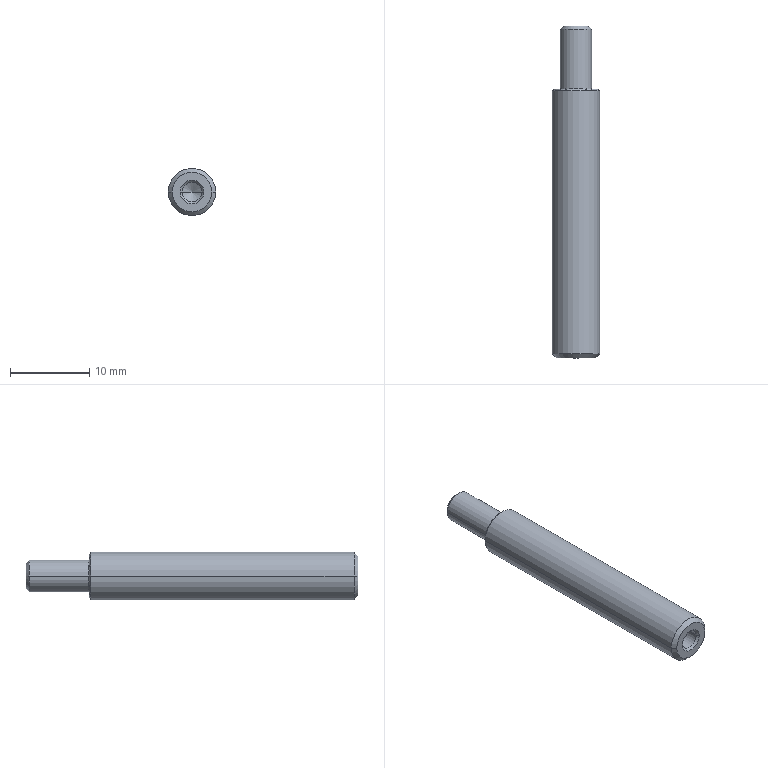Component | SolidWorks | SGE14-D6-L34-F8-B6-P4-N3-1 | 1 solid | 21 faces | box 6 x 42 x 6 mm | volume 1025 mm3 | cone 10 | cylinder 6 | plane 3 | torus 2 | commonest cylinder face diameters 2.459 x2 6 x2 4 x2
build123d program:
from build123d import *


with BuildPart() as part:
    # Sketch1 → Revolve1 (revolve)
    with BuildSketch(Plane(origin=(0, 0, 0), x_dir=(0, 0, -1), z_dir=(1, 0, 0)), mode=Mode.PRIVATE) as revolve1_sk:
        with BuildLine():
            Line((0, 0), (0, 2.5))
            Line((0, 2.5), (0.5, 3))
            Line((0.5, 3), (33.8, 3))
            Line((33.8, 3), (34, 2.8))
            Line((34, 2.8), (34, 2.1))
            ThreePointArc((34, 2.1), (34.029, 2.029), (34.1, 2))
            Line((34.1, 2), (41.571, 2))
            Line((41.571, 2), (42, 1.571))
            Line((42, 1.571), (42, 0))
            Line((42, 0), (0, 0))
        make_face()
    revolve(revolve1_sk.sketch.rotate(Axis((0, 0, -42), (0, 0, 1)), 270), axis=Axis((0, 0, -42), (0, 0, 1)))

    # Sketch2 → Cut-Revolve1 (revolve, cut)
    with BuildSketch(Plane(origin=(0, 0, 0), x_dir=(0, 0, -1), z_dir=(1, 0, 0)), mode=Mode.PRIVATE) as cut_revolve1_sk:
        Polygon((0, 0), (0, 1.5), (0.2705, 1.23), (6.656, 1.23), (7.366, 0), align=None)
    revolve(cut_revolve1_sk.sketch.rotate(Axis((0, 0, -7.366), (0, 0, 1)), 270), axis=Axis((0, 0, -7.366), (0, 0, 1)), mode=Mode.SUBTRACT)


solid = part.part

# Placed as in the assembly
solid = solid.moved(Location((-57.536, 39.25, 217.788), (90, 0, 0)))
STEP:
#1=COLOUR_RGB('',0.7922,0.8196,0.9333);
#2=FILL_AREA_STYLE_COLOUR('',#1);
#3=FILL_AREA_STYLE('',(#2));
#4=SURFACE_STYLE_FILL_AREA(#3);
#5=SURFACE_SIDE_STYLE('',(#4));
#6=SURFACE_STYLE_USAGE(.BOTH.,#5);
#7=PRESENTATION_STYLE_ASSIGNMENT((#6));
#8=CARTESIAN_POINT('',(-2.265,1.835,8.574));
#9=VERTEX_POINT('',#8);
#10=CARTESIAN_POINT('',(-2.217,1.807,8.574));
#11=VERTEX_POINT('',#10);
#12=CARTESIAN_POINT('',(-2.265,1.835,8.574));
#13=DIRECTION('',(0.866,-0.5,-0.));
#14=VECTOR('',#13,39.37);
#15=LINE('',#12,#14);
#16=EDGE_CURVE('',#9,#11,#15,.T.);
#17=ORIENTED_EDGE('',*,*,#16,.F.);
#18=CARTESIAN_POINT('',(-2.314,1.807,8.574));
#19=VERTEX_POINT('',#18);
#20=CARTESIAN_POINT('',(-2.265,1.835,8.574));
#21=DIRECTION('',(-0.866,-0.5,0.));
#22=VECTOR('',#21,39.37);
#23=LINE('',#20,#22);
#24=EDGE_CURVE('',#9,#19,#23,.T.);
#25=ORIENTED_EDGE('',*,*,#24,.T.);
#26=CARTESIAN_POINT('',(-2.265,1.807,8.574));
#27=DIRECTION('',(0.,-1.,-0.));
#28=DIRECTION('',(1.,0.,0.));
#29=AXIS2_PLACEMENT_3D('',#26,#27,#28);
#30=CIRCLE('',#29,0.04841);
#31=EDGE_CURVE('',#19,#11,#30,.T.);
#32=ORIENTED_EDGE('',*,*,#31,.T.);
#33=EDGE_LOOP('',(#17,#25,#32));
#34=FACE_OUTER_BOUND('',#33,.T.);
#35=CARTESIAN_POINT('',(-2.265,-37.535,8.574));
#36=DIRECTION('',(0.,-1.,-0.));
#37=DIRECTION('',(1.,0.,-0.));
#38=AXIS2_PLACEMENT_3D('',#35,#36,#37);
#39=CONICAL_SURFACE('',#38,68.191,1.047);
#40=ADVANCED_FACE('',(#34),#39,.F.);
#41=ORIENTED_EDGE('',*,*,#31,.F.);
#42=CARTESIAN_POINT('',(-2.314,1.556,8.574));
#43=VERTEX_POINT('',#42);
#44=CARTESIAN_POINT('',(-2.314,1.835,8.574));
#45=DIRECTION('',(0.,-1.,-0.));
#46=VECTOR('',#45,39.37);
#47=LINE('',#44,#46);
#48=EDGE_CURVE('',#19,#43,#47,.T.);
#49=ORIENTED_EDGE('',*,*,#48,.T.);
#50=CARTESIAN_POINT('',(-2.217,1.556,8.574));
#51=VERTEX_POINT('',#50);
#52=CARTESIAN_POINT('',(-2.265,1.556,8.574));
#53=DIRECTION('',(0.,-1.,-0.));
#54=DIRECTION('',(1.,0.,0.));
#55=AXIS2_PLACEMENT_3D('',#52,#53,#54);
#56=CIRCLE('',#55,0.04841);
#57=EDGE_CURVE('',#43,#51,#56,.T.);
#58=ORIENTED_EDGE('',*,*,#57,.T.);
#59=CARTESIAN_POINT('',(-2.217,1.835,8.574));
#60=DIRECTION('',(0.,-1.,-0.));
#61=VECTOR('',#60,39.37);
#62=LINE('',#59,#61);
#63=EDGE_CURVE('',#11,#51,#62,.T.);
#64=ORIENTED_EDGE('',*,*,#63,.F.);
#65=EDGE_LOOP('',(#41,#49,#58,#64));
#66=FACE_OUTER_BOUND('',#65,.T.);
#67=CARTESIAN_POINT('',(-2.265,1.835,8.574));
#68=DIRECTION('',(0.,-1.,-0.));
#69=DIRECTION('',(1.,0.,0.));
#70=AXIS2_PLACEMENT_3D('',#67,#68,#69);
#71=CYLINDRICAL_SURFACE('',#70,0.04841);
#72=ADVANCED_FACE('',(#66),#71,.F.);
#73=ORIENTED_EDGE('',*,*,#57,.F.);
#74=CARTESIAN_POINT('',(-2.324,1.545,8.574));
#75=VERTEX_POINT('',#74);
#76=CARTESIAN_POINT('',(-2.314,1.556,8.574));
#77=DIRECTION('',(-0.7071,-0.7071,0.));
#78=VECTOR('',#77,39.37);
#79=LINE('',#76,#78);
#80=EDGE_CURVE('',#43,#75,#79,.T.);
#81=ORIENTED_EDGE('',*,*,#80,.T.);
#82=CARTESIAN_POINT('',(-2.206,1.545,8.574));
#83=VERTEX_POINT('',#82);
#84=CARTESIAN_POINT('',(-2.265,1.545,8.574));
#85=DIRECTION('',(0.,-1.,-0.));
#86=DIRECTION('',(1.,0.,0.));
#87=AXIS2_PLACEMENT_3D('',#84,#85,#86);
#88=CIRCLE('',#87,0.05906);
#89=EDGE_CURVE('',#75,#83,#88,.T.);
#90=ORIENTED_EDGE('',*,*,#89,.T.);
#91=CARTESIAN_POINT('',(-2.217,1.556,8.574));
#92=DIRECTION('',(0.7071,-0.7071,-0.));
#93=VECTOR('',#92,39.37);
#94=LINE('',#91,#93);
#95=EDGE_CURVE('',#51,#83,#94,.T.);
#96=ORIENTED_EDGE('',*,*,#95,.F.);
#97=EDGE_LOOP('',(#73,#81,#90,#96));
#98=FACE_OUTER_BOUND('',#97,.T.);
#99=CARTESIAN_POINT('',(-2.265,1.556,8.574));
#100=DIRECTION('',(0.,-1.,-0.));
#101=DIRECTION('',(1.,0.,0.));
#102=AXIS2_PLACEMENT_3D('',#99,#100,#101);
#103=CONICAL_SURFACE('',#102,0.04841,0.7854);
#104=ADVANCED_FACE('',(#98),#103,.F.);
#105=CARTESIAN_POINT('',(-2.167,1.545,8.574));
#106=VERTEX_POINT('',#105);
#107=CARTESIAN_POINT('',(-2.364,1.545,8.574));
#108=VERTEX_POINT('',#107);
#109=CARTESIAN_POINT('',(-2.265,1.545,8.574));
#110=DIRECTION('',(0.,-1.,-0.));
#111=DIRECTION('',(1.,0.,0.));
#112=AXIS2_PLACEMENT_3D('',#109,#110,#111);
#113=CIRCLE('',#112,0.09843);
#114=EDGE_CURVE('',#106,#108,#113,.T.);
#115=ORIENTED_EDGE('',*,*,#114,.F.);
#116=CARTESIAN_POINT('',(-2.147,1.565,8.574));
#117=VERTEX_POINT('',#116);
#118=CARTESIAN_POINT('',(-2.147,1.565,8.574));
#119=DIRECTION('',(0.7071,0.7071,0.));
#120=VECTOR('',#119,39.37);
#121=LINE('',#118,#120);
#122=EDGE_CURVE('',#106,#117,#121,.T.);
#123=ORIENTED_EDGE('',*,*,#122,.T.);
#124=CARTESIAN_POINT('',(-2.383,1.565,8.574));
#125=VERTEX_POINT('',#124);
#126=CARTESIAN_POINT('',(-2.265,1.565,8.574));
#127=DIRECTION('',(0.,-1.,-0.));
#128=DIRECTION('',(1.,0.,0.));
#129=AXIS2_PLACEMENT_3D('',#126,#127,#128);
#130=CIRCLE('',#129,0.1181);
#131=EDGE_CURVE('',#117,#125,#130,.T.);
#132=ORIENTED_EDGE('',*,*,#131,.T.);
#133=CARTESIAN_POINT('',(-2.383,1.565,8.574));
#134=DIRECTION('',(-0.7071,0.7071,0.));
#135=VECTOR('',#134,39.37);
#136=LINE('',#133,#135);
#137=EDGE_CURVE('',#108,#125,#136,.T.);
#138=ORIENTED_EDGE('',*,*,#137,.F.);
#139=EDGE_LOOP('',(#115,#123,#132,#138));
#140=FACE_OUTER_BOUND('',#139,.T.);
#141=CARTESIAN_POINT('',(-2.265,1.565,8.574));
#142=DIRECTION('',(-0.,1.,0.));
#143=DIRECTION('',(-1.,0.,0.));
#144=AXIS2_PLACEMENT_3D('',#141,#142,#143);
#145=CONICAL_SURFACE('',#144,0.1181,0.7854);
#146=ADVANCED_FACE('',(#140),#145,.T.);
#147=CARTESIAN_POINT('',(-2.147,2.876,8.574));
#148=VERTEX_POINT('',#147);
#149=CARTESIAN_POINT('',(-2.383,2.876,8.574));
#150=VERTEX_POINT('',#149);
#151=CARTESIAN_POINT('',(-2.265,2.876,8.574));
#152=DIRECTION('',(0.,-1.,-0.));
#153=DIRECTION('',(1.,0.,0.));
#154=AXIS2_PLACEMENT_3D('',#151,#152,#153);
#155=CIRCLE('',#154,0.1181);
#156=EDGE_CURVE('',#148,#150,#155,.T.);
#157=ORIENTED_EDGE('',*,*,#156,.T.);
#158=CARTESIAN_POINT('',(-2.383,3.199,8.574));
#159=DIRECTION('',(0.,-1.,-0.));
#160=VECTOR('',#159,39.37);
#161=LINE('',#158,#160);
#162=EDGE_CURVE('',#150,#125,#161,.T.);
#163=ORIENTED_EDGE('',*,*,#162,.T.);
#164=ORIENTED_EDGE('',*,*,#131,.F.);
#165=CARTESIAN_POINT('',(-2.147,3.199,8.574));
#166=DIRECTION('',(0.,-1.,-0.));
#167=VECTOR('',#166,39.37);
#168=LINE('',#165,#167);
#169=EDGE_CURVE('',#148,#117,#168,.T.);
#170=ORIENTED_EDGE('',*,*,#169,.F.);
#171=EDGE_LOOP('',(#157,#163,#164,#170));
#172=FACE_OUTER_BOUND('',#171,.T.);
#173=CARTESIAN_POINT('',(-2.265,3.199,8.574));
#174=DIRECTION('',(0.,-1.,-0.));
#175=DIRECTION('',(1.,0.,0.));
#176=AXIS2_PLACEMENT_3D('',#173,#174,#175);
#177=CYLINDRICAL_SURFACE('',#176,0.1181);
#178=ADVANCED_FACE('',(#172),#177,.T.);
#179=CARTESIAN_POINT('',(-2.155,2.884,8.574));
#180=VERTEX_POINT('',#179);
#181=CARTESIAN_POINT('',(-2.375,2.884,8.574));
#182=VERTEX_POINT('',#181);
#183=CARTESIAN_POINT('',(-2.265,2.884,8.574));
#184=DIRECTION('',(0.,-1.,-0.));
#185=DIRECTION('',(1.,0.,0.));
#186=AXIS2_PLACEMENT_3D('',#183,#184,#185);
#187=CIRCLE('',#186,0.1102);
#188=EDGE_CURVE('',#180,#182,#187,.T.);
#189=ORIENTED_EDGE('',*,*,#188,.T.);
#190=CARTESIAN_POINT('',(-2.375,2.884,8.574));
#191=DIRECTION('',(-0.7071,-0.7071,0.));
#192=VECTOR('',#191,39.37);
#193=LINE('',#190,#192);
#194=EDGE_CURVE('',#182,#150,#193,.T.);
#195=ORIENTED_EDGE('',*,*,#194,.T.);
#196=ORIENTED_EDGE('',*,*,#156,.F.);
#197=CARTESIAN_POINT('',(-2.155,2.884,8.574));
#198=DIRECTION('',(0.7071,-0.7071,-0.));
#199=VECTOR('',#198,39.37);
#200=LINE('',#197,#199);
#201=EDGE_CURVE('',#180,#148,#200,.T.);
#202=ORIENTED_EDGE('',*,*,#201,.F.);
#203=EDGE_LOOP('',(#189,#195,#196,#202));
#204=FACE_OUTER_BOUND('',#203,.T.);
#205=CARTESIAN_POINT('',(-2.265,2.884,8.574));
#206=DIRECTION('',(0.,-1.,-0.));
#207=DIRECTION('',(1.,0.,0.));
#208=AXIS2_PLACEMENT_3D('',#205,#206,#207);
#209=CONICAL_SURFACE('',#208,0.1102,0.7854);
#210=ADVANCED_FACE('',(#204),#209,.T.);
#211=CARTESIAN_POINT('',(-2.348,2.884,8.574));
#212=VERTEX_POINT('',#211);
#213=CARTESIAN_POINT('',(-2.183,2.884,8.574));
#214=VERTEX_POINT('',#213);
#215=CARTESIAN_POINT('',(-2.265,2.884,8.574));
#216=DIRECTION('',(0.,-1.,-0.));
#217=DIRECTION('',(1.,0.,0.));
#218=AXIS2_PLACEMENT_3D('',#215,#216,#217);
#219=CIRCLE('',#218,0.08268);
#220=EDGE_CURVE('',#212,#214,#219,.T.);
#221=ORIENTED_EDGE('',*,*,#220,.F.);
#222=CARTESIAN_POINT('',(-2.344,2.888,8.574));
#223=VERTEX_POINT('',#222);
#224=CARTESIAN_POINT('',(-2.348,2.888,8.574));
#225=DIRECTION('',(0.,-0.,1.));
#226=DIRECTION('',(1.,0.,0.));
#227=AXIS2_PLACEMENT_3D('',#224,#225,#226);
#228=CIRCLE('',#227,0.003937);
#229=EDGE_CURVE('',#212,#223,#228,.T.);
#230=ORIENTED_EDGE('',*,*,#229,.T.);
#231=CARTESIAN_POINT('',(-2.186,2.888,8.574));
#232=VERTEX_POINT('',#231);
#233=CARTESIAN_POINT('',(-2.265,2.888,8.574));
#234=DIRECTION('',(0.,-1.,-0.));
#235=DIRECTION('',(1.,0.,0.));
#236=AXIS2_PLACEMENT_3D('',#233,#234,#235);
#237=CIRCLE('',#236,0.07874);
#238=EDGE_CURVE('',#223,#232,#237,.T.);
#239=ORIENTED_EDGE('',*,*,#238,.T.);
#240=CARTESIAN_POINT('',(-2.183,2.888,8.574));
#241=DIRECTION('',(-0.,0.,-1.));
#242=DIRECTION('',(0.,1.,0.));
#243=AXIS2_PLACEMENT_3D('',#240,#241,#242);
#244=CIRCLE('',#243,0.003937);
#245=EDGE_CURVE('',#214,#232,#244,.T.);
#246=ORIENTED_EDGE('',*,*,#245,.F.);
#247=EDGE_LOOP('',(#221,#230,#239,#246));
#248=FACE_OUTER_BOUND('',#247,.T.);
#249=CARTESIAN_POINT('',(-2.265,2.888,8.574));
#250=DIRECTION('',(0.,-1.,-0.));
#251=DIRECTION('',(1.,0.,0.));
#252=AXIS2_PLACEMENT_3D('',#249,#250,#251);
#253=TOROIDAL_SURFACE('',#252,0.08268,0.003937);
#254=ADVANCED_FACE('',(#248),#253,.F.);
#255=CARTESIAN_POINT('',(-2.186,3.182,8.574));
#256=VERTEX_POINT('',#255);
#257=CARTESIAN_POINT('',(-2.344,3.182,8.574));
#258=VERTEX_POINT('',#257);
#259=CARTESIAN_POINT('',(-2.265,3.182,8.574));
#260=DIRECTION('',(0.,-1.,-0.));
#261=DIRECTION('',(1.,0.,0.));
#262=AXIS2_PLACEMENT_3D('',#259,#260,#261);
#263=CIRCLE('',#262,0.07874);
#264=EDGE_CURVE('',#256,#258,#263,.T.);
#265=ORIENTED_EDGE('',*,*,#264,.T.);
#266=CARTESIAN_POINT('',(-2.344,3.199,8.574));
#267=DIRECTION('',(0.,-1.,-0.));
#268=VECTOR('',#267,39.37);
#269=LINE('',#266,#268);
#270=EDGE_CURVE('',#258,#223,#269,.T.);
#271=ORIENTED_EDGE('',*,*,#270,.T.);
#272=CARTESIAN_POINT('',(-2.265,2.888,8.574));
#273=DIRECTION('',(0.,-1.,-0.));
#274=DIRECTION('',(1.,0.,0.));
#275=AXIS2_PLACEMENT_3D('',#272,#273,#274);
#276=CIRCLE('',#275,0.07874);
#277=EDGE_CURVE('',#232,#223,#276,.T.);
#278=ORIENTED_EDGE('',*,*,#277,.F.);
#279=CARTESIAN_POINT('',(-2.186,3.199,8.574));
#280=DIRECTION('',(0.,-1.,-0.));
#281=VECTOR('',#280,39.37);
#282=LINE('',#279,#281);
#283=EDGE_CURVE('',#256,#232,#282,.T.);
#284=ORIENTED_EDGE('',*,*,#283,.F.);
#285=EDGE_LOOP('',(#265,#271,#278,#284));
#286=FACE_OUTER_BOUND('',#285,.T.);
#287=CARTESIAN_POINT('',(-2.265,3.199,8.574));
#288=DIRECTION('',(0.,-1.,-0.));
#289=DIRECTION('',(1.,0.,0.));
#290=AXIS2_PLACEMENT_3D('',#287,#288,#289);
#291=CYLINDRICAL_SURFACE('',#290,0.07874);
#292=ADVANCED_FACE('',(#286),#291,.T.);
#293=CARTESIAN_POINT('',(-2.203,3.199,8.574));
#294=VERTEX_POINT('',#293);
#295=CARTESIAN_POINT('',(-2.327,3.199,8.574));
#296=VERTEX_POINT('',#295);
#297=CARTESIAN_POINT('',(-2.265,3.199,8.574));
#298=DIRECTION('',(0.,-1.,-0.));
#299=DIRECTION('',(1.,0.,0.));
#300=AXIS2_PLACEMENT_3D('',#297,#298,#299);
#301=CIRCLE('',#300,0.06183);
#302=EDGE_CURVE('',#294,#296,#301,.T.);
#303=ORIENTED_EDGE('',*,*,#302,.T.);
#304=CARTESIAN_POINT('',(-2.327,3.199,8.574));
#305=DIRECTION('',(-0.7071,-0.7071,0.));
#306=VECTOR('',#305,39.37);
#307=LINE('',#304,#306);
#308=EDGE_CURVE('',#296,#258,#307,.T.);
#309=ORIENTED_EDGE('',*,*,#308,.T.);
#310=ORIENTED_EDGE('',*,*,#264,.F.);
#311=CARTESIAN_POINT('',(-2.203,3.199,8.574));
#312=DIRECTION('',(0.7071,-0.7071,-0.));
#313=VECTOR('',#312,39.37);
#314=LINE('',#311,#313);
#315=EDGE_CURVE('',#294,#256,#314,.T.);
#316=ORIENTED_EDGE('',*,*,#315,.F.);
#317=EDGE_LOOP('',(#303,#309,#310,#316));
#318=FACE_OUTER_BOUND('',#317,.T.);
#319=CARTESIAN_POINT('',(-2.265,3.199,8.574));
#320=DIRECTION('',(0.,-1.,-0.));
#321=DIRECTION('',(1.,0.,0.));
#322=AXIS2_PLACEMENT_3D('',#319,#320,#321);
#323=CONICAL_SURFACE('',#322,0.06183,0.7854);
#324=ADVANCED_FACE('',(#318),#323,.T.);
#325=ORIENTED_EDGE('',*,*,#302,.F.);
#326=CARTESIAN_POINT('',(-2.265,3.199,8.574));
#327=DIRECTION('',(0.,-1.,-0.));
#328=DIRECTION('',(1.,0.,0.));
#329=AXIS2_PLACEMENT_3D('',#326,#327,#328);
#330=CIRCLE('',#329,0.06183);
#331=EDGE_CURVE('',#296,#294,#330,.T.);
#332=ORIENTED_EDGE('',*,*,#331,.F.);
#333=EDGE_LOOP('',(#325,#332));
#334=FACE_OUTER_BOUND('',#333,.T.);
#335=CARTESIAN_POINT('',(-2.265,3.199,8.636));
#336=DIRECTION('',(0.,-1.,-0.));
#337=DIRECTION('',(1.,0.,-0.));
#338=AXIS2_PLACEMENT_3D('',#335,#336,#337);
#339=PLANE('',#338);
#340=ADVANCED_FACE('',(#334),#339,.F.);
#341=ORIENTED_EDGE('',*,*,#308,.F.);
#342=ORIENTED_EDGE('',*,*,#331,.T.);
#343=ORIENTED_EDGE('',*,*,#315,.T.);
#344=CARTESIAN_POINT('',(-2.265,3.182,8.574));
#345=DIRECTION('',(0.,-1.,-0.));
#346=DIRECTION('',(1.,0.,0.));
#347=AXIS2_PLACEMENT_3D('',#344,#345,#346);
#348=CIRCLE('',#347,0.07874);
#349=EDGE_CURVE('',#258,#256,#348,.T.);
#350=ORIENTED_EDGE('',*,*,#349,.F.);
#351=EDGE_LOOP('',(#341,#342,#343,#350));
#352=FACE_OUTER_BOUND('',#351,.T.);
#353=CARTESIAN_POINT('',(-2.265,3.199,8.574));
#354=DIRECTION('',(0.,-1.,-0.));
#355=DIRECTION('',(1.,0.,0.));
#356=AXIS2_PLACEMENT_3D('',#353,#354,#355);
#357=CONICAL_SURFACE('',#356,0.06183,0.7854);
#358=ADVANCED_FACE('',(#352),#357,.T.);
#359=ORIENTED_EDGE('',*,*,#270,.F.);
#360=ORIENTED_EDGE('',*,*,#349,.T.);
#361=ORIENTED_EDGE('',*,*,#283,.T.);
#362=ORIENTED_EDGE('',*,*,#238,.F.);
#363=EDGE_LOOP('',(#359,#360,#361,#362));
#364=FACE_OUTER_BOUND('',#363,.T.);
#365=CARTESIAN_POINT('',(-2.265,3.199,8.574));
#366=DIRECTION('',(0.,-1.,-0.));
#367=DIRECTION('',(1.,0.,0.));
#368=AXIS2_PLACEMENT_3D('',#365,#366,#367);
#369=CYLINDRICAL_SURFACE('',#368,0.07874);
#370=ADVANCED_FACE('',(#364),#369,.T.);
#371=ORIENTED_EDGE('',*,*,#229,.F.);
#372=CARTESIAN_POINT('',(-2.265,2.884,8.574));
#373=DIRECTION('',(0.,-1.,-0.));
#374=DIRECTION('',(1.,0.,0.));
#375=AXIS2_PLACEMENT_3D('',#372,#373,#374);
#376=CIRCLE('',#375,0.08268);
#377=EDGE_CURVE('',#214,#212,#376,.T.);
#378=ORIENTED_EDGE('',*,*,#377,.F.);
#379=ORIENTED_EDGE('',*,*,#245,.T.);
#380=ORIENTED_EDGE('',*,*,#277,.T.);
#381=EDGE_LOOP('',(#371,#378,#379,#380));
#382=FACE_OUTER_BOUND('',#381,.T.);
#383=CARTESIAN_POINT('',(-2.265,2.888,8.574));
#384=DIRECTION('',(0.,-1.,-0.));
#385=DIRECTION('',(1.,0.,0.));
#386=AXIS2_PLACEMENT_3D('',#383,#384,#385);
#387=TOROIDAL_SURFACE('',#386,0.08268,0.003937);
#388=ADVANCED_FACE('',(#382),#387,.F.);
#389=ORIENTED_EDGE('',*,*,#188,.F.);
#390=CARTESIAN_POINT('',(-2.265,2.884,8.574));
#391=DIRECTION('',(0.,-1.,-0.));
#392=DIRECTION('',(1.,0.,0.));
#393=AXIS2_PLACEMENT_3D('',#390,#391,#392);
#394=CIRCLE('',#393,0.1102);
#395=EDGE_CURVE('',#182,#180,#394,.T.);
#396=ORIENTED_EDGE('',*,*,#395,.F.);
#397=EDGE_LOOP('',(#389,#396));
#398=FACE_OUTER_BOUND('',#397,.T.);
#399=ORIENTED_EDGE('',*,*,#377,.T.);
#400=ORIENTED_EDGE('',*,*,#220,.T.);
#401=EDGE_LOOP('',(#399,#400));
#402=FACE_BOUND('',#401,.T.);
#403=CARTESIAN_POINT('',(-2.265,2.884,8.685));
#404=DIRECTION('',(0.,-1.,-0.));
#405=DIRECTION('',(1.,0.,-0.));
#406=AXIS2_PLACEMENT_3D('',#403,#404,#405);
#407=PLANE('',#406);
#408=ADVANCED_FACE('',(#398,#402),#407,.F.);
#409=ORIENTED_EDGE('',*,*,#194,.F.);
#410=ORIENTED_EDGE('',*,*,#395,.T.);
#411=ORIENTED_EDGE('',*,*,#201,.T.);
#412=CARTESIAN_POINT('',(-2.265,2.876,8.574));
#413=DIRECTION('',(0.,-1.,-0.));
#414=DIRECTION('',(1.,0.,0.));
#415=AXIS2_PLACEMENT_3D('',#412,#413,#414);
#416=CIRCLE('',#415,0.1181);
#417=EDGE_CURVE('',#150,#148,#416,.T.);
#418=ORIENTED_EDGE('',*,*,#417,.F.);
#419=EDGE_LOOP('',(#409,#410,#411,#418));
#420=FACE_OUTER_BOUND('',#419,.T.);
#421=CARTESIAN_POINT('',(-2.265,2.884,8.574));
#422=DIRECTION('',(0.,-1.,-0.));
#423=DIRECTION('',(1.,0.,0.));
#424=AXIS2_PLACEMENT_3D('',#421,#422,#423);
#425=CONICAL_SURFACE('',#424,0.1102,0.7854);
#426=ADVANCED_FACE('',(#420),#425,.T.);
#427=ORIENTED_EDGE('',*,*,#162,.F.);
#428=ORIENTED_EDGE('',*,*,#417,.T.);
#429=ORIENTED_EDGE('',*,*,#169,.T.);
#430=CARTESIAN_POINT('',(-2.265,1.565,8.574));
#431=DIRECTION('',(0.,-1.,-0.));
#432=DIRECTION('',(1.,0.,0.));
#433=AXIS2_PLACEMENT_3D('',#430,#431,#432);
#434=CIRCLE('',#433,0.1181);
#435=EDGE_CURVE('',#125,#117,#434,.T.);
#436=ORIENTED_EDGE('',*,*,#435,.F.);
#437=EDGE_LOOP('',(#427,#428,#429,#436));
#438=FACE_OUTER_BOUND('',#437,.T.);
#439=CARTESIAN_POINT('',(-2.265,3.199,8.574));
#440=DIRECTION('',(0.,-1.,-0.));
#441=DIRECTION('',(1.,0.,0.));
#442=AXIS2_PLACEMENT_3D('',#439,#440,#441);
#443=CYLINDRICAL_SURFACE('',#442,0.1181);
#444=ADVANCED_FACE('',(#438),#443,.T.);
#445=ORIENTED_EDGE('',*,*,#122,.F.);
#446=CARTESIAN_POINT('',(-2.265,1.545,8.574));
#447=DIRECTION('',(0.,-1.,-0.));
#448=DIRECTION('',(1.,0.,0.));
#449=AXIS2_PLACEMENT_3D('',#446,#447,#448);
#450=CIRCLE('',#449,0.09843);
#451=EDGE_CURVE('',#108,#106,#450,.T.);
#452=ORIENTED_EDGE('',*,*,#451,.F.);
#453=ORIENTED_EDGE('',*,*,#137,.T.);
#454=ORIENTED_EDGE('',*,*,#435,.T.);
#455=EDGE_LOOP('',(#445,#452,#453,#454));
#456=FACE_OUTER_BOUND('',#455,.T.);
#457=CARTESIAN_POINT('',(-2.265,1.565,8.574));
#458=DIRECTION('',(-0.,1.,0.));
#459=DIRECTION('',(-1.,0.,0.));
#460=AXIS2_PLACEMENT_3D('',#457,#458,#459);
#461=CONICAL_SURFACE('',#460,0.1181,0.7854);
#462=ADVANCED_FACE('',(#456),#461,.T.);
#463=CARTESIAN_POINT('',(-2.265,1.545,8.574));
#464=DIRECTION('',(0.,-1.,-0.));
#465=DIRECTION('',(1.,0.,0.));
#466=AXIS2_PLACEMENT_3D('',#463,#464,#465);
#467=CIRCLE('',#466,0.05906);
#468=EDGE_CURVE('',#83,#75,#467,.T.);
#469=ORIENTED_EDGE('',*,*,#468,.F.);
#470=ORIENTED_EDGE('',*,*,#89,.F.);
#471=EDGE_LOOP('',(#469,#470));
#472=FACE_BOUND('',#471,.T.);
#473=ORIENTED_EDGE('',*,*,#451,.T.);
#474=ORIENTED_EDGE('',*,*,#114,.T.);
#475=EDGE_LOOP('',(#473,#474));
#476=FACE_OUTER_BOUND('',#475,.T.);
#477=CARTESIAN_POINT('',(-2.265,1.545,8.574));
#478=DIRECTION('',(-0.,1.,0.));
#479=DIRECTION('',(-1.,-0.,0.));
#480=AXIS2_PLACEMENT_3D('',#477,#478,#479);
#481=PLANE('',#480);
#482=ADVANCED_FACE('',(#472,#476),#481,.F.);
#483=ORIENTED_EDGE('',*,*,#80,.F.);
#484=CARTESIAN_POINT('',(-2.265,1.556,8.574));
#485=DIRECTION('',(0.,-1.,-0.));
#486=DIRECTION('',(1.,0.,0.));
#487=AXIS2_PLACEMENT_3D('',#484,#485,#486);
#488=CIRCLE('',#487,0.04841);
#489=EDGE_CURVE('',#51,#43,#488,.T.);
#490=ORIENTED_EDGE('',*,*,#489,.F.);
#491=ORIENTED_EDGE('',*,*,#95,.T.);
#492=ORIENTED_EDGE('',*,*,#468,.T.);
#493=EDGE_LOOP('',(#483,#490,#491,#492));
#494=FACE_OUTER_BOUND('',#493,.T.);
#495=CARTESIAN_POINT('',(-2.265,1.556,8.574));
#496=DIRECTION('',(0.,-1.,-0.));
#497=DIRECTION('',(1.,0.,0.));
#498=AXIS2_PLACEMENT_3D('',#495,#496,#497);
#499=CONICAL_SURFACE('',#498,0.04841,0.7854);
#500=ADVANCED_FACE('',(#494),#499,.F.);
#501=ORIENTED_EDGE('',*,*,#48,.F.);
#502=CARTESIAN_POINT('',(-2.265,1.807,8.574));
#503=DIRECTION('',(0.,-1.,-0.));
#504=DIRECTION('',(1.,0.,0.));
#505=AXIS2_PLACEMENT_3D('',#502,#503,#504);
#506=CIRCLE('',#505,0.04841);
#507=EDGE_CURVE('',#11,#19,#506,.T.);
#508=ORIENTED_EDGE('',*,*,#507,.F.);
#509=ORIENTED_EDGE('',*,*,#63,.T.);
#510=ORIENTED_EDGE('',*,*,#489,.T.);
#511=EDGE_LOOP('',(#501,#508,#509,#510));
#512=FACE_OUTER_BOUND('',#511,.T.);
#513=CARTESIAN_POINT('',(-2.265,1.835,8.574));
#514=DIRECTION('',(0.,-1.,-0.));
#515=DIRECTION('',(1.,0.,0.));
#516=AXIS2_PLACEMENT_3D('',#513,#514,#515);
#517=CYLINDRICAL_SURFACE('',#516,0.04841);
#518=ADVANCED_FACE('',(#512),#517,.F.);
#519=ORIENTED_EDGE('',*,*,#24,.F.);
#520=ORIENTED_EDGE('',*,*,#16,.T.);
#521=ORIENTED_EDGE('',*,*,#507,.T.);
#522=EDGE_LOOP('',(#519,#520,#521));
#523=FACE_OUTER_BOUND('',#522,.T.);
#524=CARTESIAN_POINT('',(-2.265,-37.535,8.574));
#525=DIRECTION('',(0.,-1.,-0.));
#526=DIRECTION('',(1.,0.,-0.));
#527=AXIS2_PLACEMENT_3D('',#524,#525,#526);
#528=CONICAL_SURFACE('',#527,68.191,1.047);
#529=ADVANCED_FACE('',(#523),#528,.F.);
#530=CLOSED_SHELL('',(#40,#72,#104,#146,#178,#210,#254,#292,#324,#340,#358,#370,#388,#408,#426,#444,#462,#482,#500,#518,#529));
#531=MANIFOLD_SOLID_BREP('',#530);
#532=STYLED_ITEM('',(#7),#531);
#533=(LENGTH_UNIT()NAMED_UNIT(*)SI_UNIT($,.METRE.));
#534=LENGTH_MEASURE_WITH_UNIT(LENGTH_MEASURE(0.0254),#533);
#535=DIMENSIONAL_EXPONENTS(1.,0.,0.,0.,0.,0.,0.);
#536=(CONVERSION_BASED_UNIT('',#534)LENGTH_UNIT()NAMED_UNIT(#535));
#537=UNCERTAINTY_MEASURE_WITH_UNIT(LENGTH_MEASURE(0.00001),#536,'','');
#538=(NAMED_UNIT(*)PLANE_ANGLE_UNIT()SI_UNIT($,.RADIAN.));
#539=(NAMED_UNIT(*)SI_UNIT($,.STERADIAN.)SOLID_ANGLE_UNIT());
#540=(GEOMETRIC_REPRESENTATION_CONTEXT(3)GLOBAL_UNCERTAINTY_ASSIGNED_CONTEXT((#537))GLOBAL_UNIT_ASSIGNED_CONTEXT((#536,#538,#539))REPRESENTATION_CONTEXT('',''));
#541=MECHANICAL_DESIGN_GEOMETRIC_PRESENTATION_REPRESENTATION('',(#532),#540);
#542=PRESENTATION_LAYER_ASSIGNMENT('','',(#532));
#543=CARTESIAN_POINT('',(0.,0.,0.));
#544=DIRECTION('',(0.,0.,1.));
#545=DIRECTION('',(1.,0.,0.));
#546=AXIS2_PLACEMENT_3D('',#543,#544,#545);
#547=(LENGTH_UNIT()NAMED_UNIT(*)SI_UNIT($,.METRE.));
#548=LENGTH_MEASURE_WITH_UNIT(LENGTH_MEASURE(0.0254),#547);
#549=DIMENSIONAL_EXPONENTS(1.,0.,0.,0.,0.,0.,0.);
#550=(CONVERSION_BASED_UNIT('',#548)LENGTH_UNIT()NAMED_UNIT(#549));
#551=UNCERTAINTY_MEASURE_WITH_UNIT(LENGTH_MEASURE(0.00001),#550,'','');
#552=(NAMED_UNIT(*)PLANE_ANGLE_UNIT()SI_UNIT($,.RADIAN.));
#553=(NAMED_UNIT(*)SI_UNIT($,.STERADIAN.)SOLID_ANGLE_UNIT());
#554=(GEOMETRIC_REPRESENTATION_CONTEXT(3)GLOBAL_UNCERTAINTY_ASSIGNED_CONTEXT((#551))GLOBAL_UNIT_ASSIGNED_CONTEXT((#550,#552,#553))REPRESENTATION_CONTEXT('',''));
#555=ADVANCED_BREP_SHAPE_REPRESENTATION('',(#531,#546),#554);